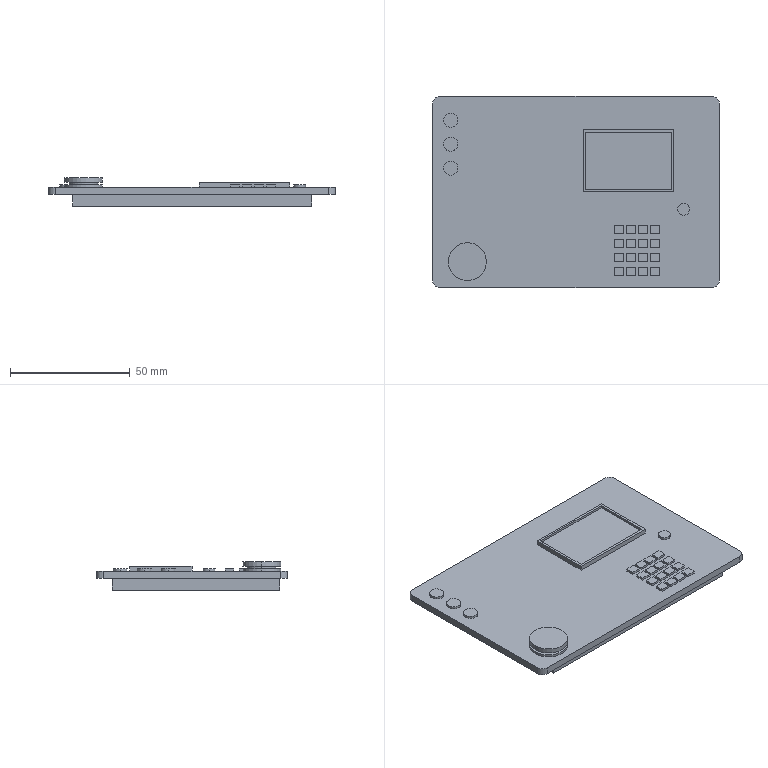Component | SolidWorks | Screen-1 | 1 solid | 126 faces | box 120 x 80 x 12 mm | volume 65922 mm3 | plane 108 | cylinder 18 | commonest cylinder face diameters 5.909 x6 15.876 x4 6 x4 12 x2 5 x2
build123d program:
from build123d import *

# Parameters (mm, degrees)
SKETCH1_W           = 100
SKETCH1_H           = 70
BOSS_EXTRUDE1_DEPTH = 5
SKETCH2_W           = 120
SKETCH2_H           = 80
BOSS_EXTRUDE2_DEPTH = 3
SKETCH4_R           = 2.5
SKETCH4_W           = 36
SKETCH4_H           = 24
SKETCH4_W_2         = 4
SKETCH4_H_2         = 3.5
BOSS_EXTRUDE3_DEPTH = 1
SKETCH5_R           = 7.938
SKETCH5_R_2         = 2.954
BOSS_EXTRUDE4_DEPTH = 1
SKETCH6_W           = 38
SKETCH6_H           = 26
SKETCH6_W_2         = 36
SKETCH6_H_2         = 24
BOSS_EXTRUDE6_DEPTH = 2
FILLET1_R           = 3
SKETCH7_R           = 6
BOSS_EXTRUDE7_DEPTH = 1
SKETCH8_R           = 7.938
BOSS_EXTRUDE8_DEPTH = 2


with BuildPart() as part:
    # Sketch1 → Boss-Extrude1 (new body)
    with BuildSketch(Plane.XY):
        with Locations((50, 35)):
            Rectangle(SKETCH1_W, SKETCH1_H)
    extrude(amount=BOSS_EXTRUDE1_DEPTH)

    # Sketch2 → Boss-Extrude2 (add)
    with BuildSketch(Plane.XY.offset(5)):
        with Locations((49.827, 36.704)):
            Rectangle(SKETCH2_W, SKETCH2_H)
    extrude(amount=BOSS_EXTRUDE2_DEPTH)

    # Sketch4 → Boss-Extrude3 (add)
    with BuildSketch(Plane.XY.offset(8)):
        with Locations((94.882, 29.505)):
            Circle(SKETCH4_R)
        with Locations((71.827, 49.704)):
            Rectangle(SKETCH4_W, SKETCH4_H)
        with Locations((72.838, 20.954)):
            Rectangle(SKETCH4_W_2, SKETCH4_H_2)
        with Locations((67.838, 20.954)):
            Rectangle(SKETCH4_W_2, SKETCH4_H_2)
        with Locations((77.838, 20.954)):
            Rectangle(SKETCH4_W_2, SKETCH4_H_2)
        with Locations((82.838, 20.954)):
            Rectangle(SKETCH4_W_2, SKETCH4_H_2)
        with Locations((67.838, 15.121)):
            Rectangle(SKETCH4_W_2, SKETCH4_H_2)
        with Locations((72.838, 15.121)):
            Rectangle(SKETCH4_W_2, SKETCH4_H_2)
        with Locations((77.838, 15.121)):
            Rectangle(SKETCH4_W_2, SKETCH4_H_2)
        with Locations((82.838, 15.121)):
            Rectangle(SKETCH4_W_2, SKETCH4_H_2)
        with Locations((67.838, 9.287)):
            Rectangle(SKETCH4_W_2, SKETCH4_H_2)
        with Locations((72.838, 9.287)):
            Rectangle(SKETCH4_W_2, SKETCH4_H_2)
        with Locations((77.838, 9.287)):
            Rectangle(SKETCH4_W_2, SKETCH4_H_2)
        with Locations((82.838, 9.287)):
            Rectangle(SKETCH4_W_2, SKETCH4_H_2)
        with Locations((67.838, 3.454)):
            Rectangle(SKETCH4_W_2, SKETCH4_H_2)
        with Locations((72.838, 3.454)):
            Rectangle(SKETCH4_W_2, SKETCH4_H_2)
        with Locations((77.838, 3.454)):
            Rectangle(SKETCH4_W_2, SKETCH4_H_2)
        with Locations((82.838, 3.454)):
            Rectangle(SKETCH4_W_2, SKETCH4_H_2)
    extrude(amount=BOSS_EXTRUDE3_DEPTH)

    # Sketch5 → Boss-Extrude4 (add)
    with BuildSketch(Plane.XY.offset(8)):
        with Locations((4.399, 7.536)):
            Circle(SKETCH5_R)
        with Locations((-2.551, 66.704)):
            Circle(SKETCH5_R_2)
        with Locations((-2.551, 56.704)):
            Circle(SKETCH5_R_2)
        with Locations((-2.551, 46.704)):
            Circle(SKETCH5_R_2)
    extrude(amount=BOSS_EXTRUDE4_DEPTH)

    # Sketch6 → Boss-Extrude6 (add)
    with BuildSketch(Plane.XY.offset(8)):
        with Locations((71.827, 49.704)):
            Rectangle(SKETCH6_W, SKETCH6_H)
        with Locations((71.827, 49.704)):
            Rectangle(SKETCH6_W_2, SKETCH6_H_2, mode=Mode.SUBTRACT)
    extrude(amount=BOSS_EXTRUDE6_DEPTH)

    # Fillet1
    fillet1_edges = [part.edges().sort_by_distance(p)[0] for p in [
        (109.827, -3.296, 6.5),
        (109.827, 76.704, 6.5),
        (-10.173, 76.704, 6.5),
        (-10.173, -3.296, 6.5),
    ]]
    fillet(fillet1_edges, radius=FILLET1_R)

    # Sketch7 → Boss-Extrude7 (add)
    with BuildSketch(Plane.XY.offset(9)):
        with Locations((4.399, 7.536)):
            Circle(SKETCH7_R)
    extrude(amount=BOSS_EXTRUDE7_DEPTH)

    # Sketch8 → Boss-Extrude8 (add)
    with BuildSketch(Plane.XY.offset(10)):
        with Locations((4.399, 7.536)):
            Circle(SKETCH8_R)
    extrude(amount=BOSS_EXTRUDE8_DEPTH)


solid = part.part

# Placed as in the assembly
solid = solid.moved(Location((-565, 118.296, 195), (0, 0, 0)))